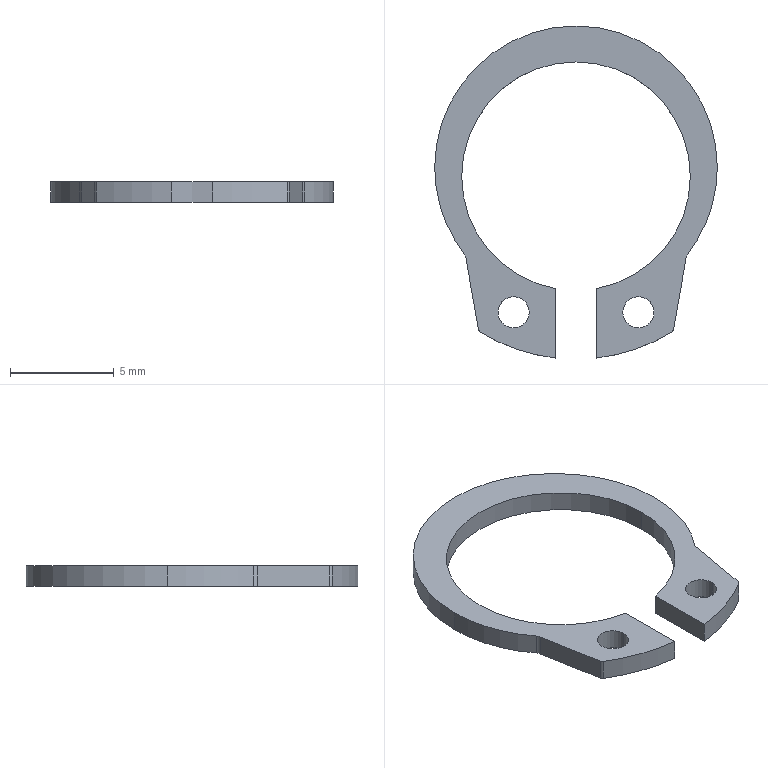Component | SolidWorks | circlips for shaft--type a large gb-1 | 1 solid | 22 faces | box 13.6 x 15.97 x 1 mm | volume 66 mm3 | cylinder 16 | plane 6 | commonest cylinder face diameters 1.5 x4 13.6 x3 11 x3 17.6 x2 0.4 x2 1 x2
build123d program:
from build123d import *

# Parameters (mm, degrees)
SKETCH1_R  = 0.75
BODY_DEPTH = 1
FILLET1_R  = 0.2
FILLET2_R  = 0.5


with BuildPart() as part:
    # Sketch1 → Body (new body)
    with BuildSketch(Plane.XY):
        with BuildLine():
            Line((-1, -5.838), (-1, -9.173))
            ThreePointArc((-1, -9.173), (-2.911, -8.734), (-4.678, -7.884))
            Line((-4.678, -7.884), (-5.322, -4.233))
            ThreePointArc((-5.322, -4.233), (0, 6.8), (5.322, -4.233))
            Line((5.322, -4.233), (4.678, -7.884))
            ThreePointArc((4.678, -7.884), (2.911, -8.734), (1, -9.173))
            Line((1, -9.173), (1, -5.838))
            ThreePointArc((1, -5.838), (0, 5.07), (-1, -5.838))
        make_face()
        with Locations(Location((3, -6.975, 0), (0, 0, 180))):
            Circle(SKETCH1_R, mode=Mode.SUBTRACT)
        with Locations((-3, -6.975)):
            Circle(SKETCH1_R, mode=Mode.SUBTRACT)
    extrude(amount=-BODY_DEPTH)

    # Fillet1
    fillet1_edges = [part.edges().sort_by_distance(p)[0] for p in [
        (-4.678, -7.884, -0.5),
        (4.678, -7.884, -0.5),
    ]]
    fillet(fillet1_edges, radius=FILLET1_R)

    # Fillet2
    fillet2_edges = [part.edges().sort_by_distance(p)[0] for p in [
        (-5.322, -4.233, -0.5),
        (5.322, -4.233, -0.5),
    ]]
    fillet(fillet2_edges, radius=FILLET2_R)


solid = part.part

# Placed as in the assembly
solid = solid.moved(Location((29.5, 189.93, 162), (0, 0, 0)))
STEP:
#1=COLOUR_RGB('',0.7922,0.8196,0.9333);
#2=FILL_AREA_STYLE_COLOUR('',#1);
#3=FILL_AREA_STYLE('',(#2));
#4=SURFACE_STYLE_FILL_AREA(#3);
#5=SURFACE_SIDE_STYLE('',(#4));
#6=SURFACE_STYLE_USAGE(.BOTH.,#5);
#7=PRESENTATION_STYLE_ASSIGNMENT((#6));
#8=CARTESIAN_POINT('',(1.25,7.203,6.339));
#9=VERTEX_POINT('',#8);
#10=CARTESIAN_POINT('',(1.309,7.203,6.339));
#11=VERTEX_POINT('',#10);
#12=CARTESIAN_POINT('',(1.28,7.203,6.339));
#13=DIRECTION('',(0.,0.,1.));
#14=DIRECTION('',(-1.,0.,0.));
#15=AXIS2_PLACEMENT_3D('',#12,#13,#14);
#16=CIRCLE('',#15,0.02953);
#17=EDGE_CURVE('',#9,#11,#16,.T.);
#18=ORIENTED_EDGE('',*,*,#17,.F.);
#19=CARTESIAN_POINT('',(1.25,7.203,6.378));
#20=VERTEX_POINT('',#19);
#21=CARTESIAN_POINT('',(1.25,7.203,6.339));
#22=DIRECTION('',(0.,0.,1.));
#23=VECTOR('',#22,39.37);
#24=LINE('',#21,#23);
#25=EDGE_CURVE('',#9,#20,#24,.T.);
#26=ORIENTED_EDGE('',*,*,#25,.T.);
#27=CARTESIAN_POINT('',(1.309,7.203,6.378));
#28=VERTEX_POINT('',#27);
#29=CARTESIAN_POINT('',(1.28,7.203,6.378));
#30=DIRECTION('',(0.,0.,1.));
#31=DIRECTION('',(-1.,0.,0.));
#32=AXIS2_PLACEMENT_3D('',#29,#30,#31);
#33=CIRCLE('',#32,0.02953);
#34=EDGE_CURVE('',#20,#28,#33,.T.);
#35=ORIENTED_EDGE('',*,*,#34,.T.);
#36=CARTESIAN_POINT('',(1.309,7.203,6.339));
#37=DIRECTION('',(0.,0.,1.));
#38=VECTOR('',#37,39.37);
#39=LINE('',#36,#38);
#40=EDGE_CURVE('',#11,#28,#39,.T.);
#41=ORIENTED_EDGE('',*,*,#40,.F.);
#42=EDGE_LOOP('',(#18,#26,#35,#41));
#43=FACE_OUTER_BOUND('',#42,.T.);
#44=CARTESIAN_POINT('',(1.28,7.203,6.339));
#45=DIRECTION('',(0.,0.,1.));
#46=DIRECTION('',(1.,0.,0.));
#47=AXIS2_PLACEMENT_3D('',#44,#45,#46);
#48=CYLINDRICAL_SURFACE('',#47,0.02953);
#49=ADVANCED_FACE('',(#43),#48,.F.);
#50=CARTESIAN_POINT('',(1.014,7.203,6.339));
#51=VERTEX_POINT('',#50);
#52=CARTESIAN_POINT('',(1.073,7.203,6.339));
#53=VERTEX_POINT('',#52);
#54=CARTESIAN_POINT('',(1.043,7.203,6.339));
#55=DIRECTION('',(0.,0.,1.));
#56=DIRECTION('',(1.,0.,0.));
#57=AXIS2_PLACEMENT_3D('',#54,#55,#56);
#58=CIRCLE('',#57,0.02953);
#59=EDGE_CURVE('',#51,#53,#58,.T.);
#60=ORIENTED_EDGE('',*,*,#59,.F.);
#61=CARTESIAN_POINT('',(1.014,7.203,6.378));
#62=VERTEX_POINT('',#61);
#63=CARTESIAN_POINT('',(1.014,7.203,6.339));
#64=DIRECTION('',(0.,0.,1.));
#65=VECTOR('',#64,39.37);
#66=LINE('',#63,#65);
#67=EDGE_CURVE('',#51,#62,#66,.T.);
#68=ORIENTED_EDGE('',*,*,#67,.T.);
#69=CARTESIAN_POINT('',(1.073,7.203,6.378));
#70=VERTEX_POINT('',#69);
#71=CARTESIAN_POINT('',(1.043,7.203,6.378));
#72=DIRECTION('',(0.,0.,1.));
#73=DIRECTION('',(1.,0.,0.));
#74=AXIS2_PLACEMENT_3D('',#71,#72,#73);
#75=CIRCLE('',#74,0.02953);
#76=EDGE_CURVE('',#62,#70,#75,.T.);
#77=ORIENTED_EDGE('',*,*,#76,.T.);
#78=CARTESIAN_POINT('',(1.073,7.203,6.339));
#79=DIRECTION('',(0.,0.,1.));
#80=VECTOR('',#79,39.37);
#81=LINE('',#78,#80);
#82=EDGE_CURVE('',#53,#70,#81,.T.);
#83=ORIENTED_EDGE('',*,*,#82,.F.);
#84=EDGE_LOOP('',(#60,#68,#77,#83));
#85=FACE_OUTER_BOUND('',#84,.T.);
#86=CARTESIAN_POINT('',(1.043,7.203,6.339));
#87=DIRECTION('',(0.,0.,1.));
#88=DIRECTION('',(1.,0.,0.));
#89=AXIS2_PLACEMENT_3D('',#86,#87,#88);
#90=CYLINDRICAL_SURFACE('',#89,0.02953);
#91=ADVANCED_FACE('',(#85),#90,.F.);
#92=CARTESIAN_POINT('',(1.429,7.478,6.339));
#93=VERTEX_POINT('',#92);
#94=CARTESIAN_POINT('',(0.8937,7.478,6.339));
#95=VERTEX_POINT('',#94);
#96=CARTESIAN_POINT('',(1.161,7.478,6.339));
#97=DIRECTION('',(0.,0.,1.));
#98=DIRECTION('',(1.,0.,0.));
#99=AXIS2_PLACEMENT_3D('',#96,#97,#98);
#100=CIRCLE('',#99,0.2677);
#101=EDGE_CURVE('',#93,#95,#100,.T.);
#102=ORIENTED_EDGE('',*,*,#101,.T.);
#103=CARTESIAN_POINT('',(0.8937,7.478,6.378));
#104=VERTEX_POINT('',#103);
#105=CARTESIAN_POINT('',(0.8937,7.478,6.339));
#106=DIRECTION('',(0.,0.,1.));
#107=VECTOR('',#106,39.37);
#108=LINE('',#105,#107);
#109=EDGE_CURVE('',#95,#104,#108,.T.);
#110=ORIENTED_EDGE('',*,*,#109,.T.);
#111=CARTESIAN_POINT('',(1.429,7.478,6.378));
#112=VERTEX_POINT('',#111);
#113=CARTESIAN_POINT('',(1.161,7.478,6.378));
#114=DIRECTION('',(0.,0.,1.));
#115=DIRECTION('',(1.,0.,0.));
#116=AXIS2_PLACEMENT_3D('',#113,#114,#115);
#117=CIRCLE('',#116,0.2677);
#118=EDGE_CURVE('',#112,#104,#117,.T.);
#119=ORIENTED_EDGE('',*,*,#118,.F.);
#120=CARTESIAN_POINT('',(1.429,7.478,6.339));
#121=DIRECTION('',(0.,0.,1.));
#122=VECTOR('',#121,39.37);
#123=LINE('',#120,#122);
#124=EDGE_CURVE('',#93,#112,#123,.T.);
#125=ORIENTED_EDGE('',*,*,#124,.F.);
#126=EDGE_LOOP('',(#102,#110,#119,#125));
#127=FACE_OUTER_BOUND('',#126,.T.);
#128=CARTESIAN_POINT('',(1.161,7.478,6.339));
#129=DIRECTION('',(0.,0.,1.));
#130=DIRECTION('',(1.,0.,0.));
#131=AXIS2_PLACEMENT_3D('',#128,#129,#130);
#132=CYLINDRICAL_SURFACE('',#131,0.2677);
#133=ADVANCED_FACE('',(#127),#132,.T.);
#134=CARTESIAN_POINT('',(1.374,7.315,6.339));
#135=VERTEX_POINT('',#134);
#136=CARTESIAN_POINT('',(1.161,7.478,6.339));
#137=DIRECTION('',(0.,0.,1.));
#138=DIRECTION('',(1.,0.,0.));
#139=AXIS2_PLACEMENT_3D('',#136,#137,#138);
#140=CIRCLE('',#139,0.2677);
#141=EDGE_CURVE('',#135,#93,#140,.T.);
#142=ORIENTED_EDGE('',*,*,#141,.T.);
#143=ORIENTED_EDGE('',*,*,#124,.T.);
#144=CARTESIAN_POINT('',(1.374,7.315,6.378));
#145=VERTEX_POINT('',#144);
#146=CARTESIAN_POINT('',(1.161,7.478,6.378));
#147=DIRECTION('',(0.,0.,1.));
#148=DIRECTION('',(1.,0.,0.));
#149=AXIS2_PLACEMENT_3D('',#146,#147,#148);
#150=CIRCLE('',#149,0.2677);
#151=EDGE_CURVE('',#145,#112,#150,.T.);
#152=ORIENTED_EDGE('',*,*,#151,.F.);
#153=CARTESIAN_POINT('',(1.374,7.315,6.339));
#154=DIRECTION('',(0.,0.,-1.));
#155=VECTOR('',#154,39.37);
#156=LINE('',#153,#155);
#157=EDGE_CURVE('',#145,#135,#156,.T.);
#158=ORIENTED_EDGE('',*,*,#157,.T.);
#159=EDGE_LOOP('',(#142,#143,#152,#158));
#160=FACE_OUTER_BOUND('',#159,.T.);
#161=CARTESIAN_POINT('',(1.161,7.478,6.339));
#162=DIRECTION('',(0.,0.,1.));
#163=DIRECTION('',(1.,0.,0.));
#164=AXIS2_PLACEMENT_3D('',#161,#162,#163);
#165=CYLINDRICAL_SURFACE('',#164,0.2677);
#166=ADVANCED_FACE('',(#160),#165,.T.);
#167=CARTESIAN_POINT('',(1.122,7.248,6.339));
#168=VERTEX_POINT('',#167);
#169=CARTESIAN_POINT('',(0.9449,7.461,6.339));
#170=VERTEX_POINT('',#169);
#171=CARTESIAN_POINT('',(1.161,7.461,6.339));
#172=DIRECTION('',(0.,0.,-1.));
#173=DIRECTION('',(1.,0.,0.));
#174=AXIS2_PLACEMENT_3D('',#171,#172,#173);
#175=CIRCLE('',#174,0.2165);
#176=EDGE_CURVE('',#168,#170,#175,.T.);
#177=ORIENTED_EDGE('',*,*,#176,.T.);
#178=CARTESIAN_POINT('',(0.9449,7.461,6.378));
#179=VERTEX_POINT('',#178);
#180=CARTESIAN_POINT('',(0.9449,7.461,6.339));
#181=DIRECTION('',(0.,0.,1.));
#182=VECTOR('',#181,39.37);
#183=LINE('',#180,#182);
#184=EDGE_CURVE('',#170,#179,#183,.T.);
#185=ORIENTED_EDGE('',*,*,#184,.T.);
#186=CARTESIAN_POINT('',(1.122,7.248,6.378));
#187=VERTEX_POINT('',#186);
#188=CARTESIAN_POINT('',(1.161,7.461,6.378));
#189=DIRECTION('',(0.,0.,-1.));
#190=DIRECTION('',(1.,0.,0.));
#191=AXIS2_PLACEMENT_3D('',#188,#189,#190);
#192=CIRCLE('',#191,0.2165);
#193=EDGE_CURVE('',#187,#179,#192,.T.);
#194=ORIENTED_EDGE('',*,*,#193,.F.);
#195=CARTESIAN_POINT('',(1.122,7.248,6.339));
#196=DIRECTION('',(0.,0.,1.));
#197=VECTOR('',#196,39.37);
#198=LINE('',#195,#197);
#199=EDGE_CURVE('',#168,#187,#198,.T.);
#200=ORIENTED_EDGE('',*,*,#199,.F.);
#201=EDGE_LOOP('',(#177,#185,#194,#200));
#202=FACE_OUTER_BOUND('',#201,.T.);
#203=CARTESIAN_POINT('',(1.161,7.461,6.339));
#204=DIRECTION('',(0.,0.,1.));
#205=DIRECTION('',(1.,0.,0.));
#206=AXIS2_PLACEMENT_3D('',#203,#204,#205);
#207=CYLINDRICAL_SURFACE('',#206,0.2165);
#208=ADVANCED_FACE('',(#202),#207,.F.);
#209=ORIENTED_EDGE('',*,*,#184,.F.);
#210=CARTESIAN_POINT('',(1.378,7.461,6.339));
#211=VERTEX_POINT('',#210);
#212=CARTESIAN_POINT('',(1.161,7.461,6.339));
#213=DIRECTION('',(0.,0.,-1.));
#214=DIRECTION('',(1.,0.,0.));
#215=AXIS2_PLACEMENT_3D('',#212,#213,#214);
#216=CIRCLE('',#215,0.2165);
#217=EDGE_CURVE('',#170,#211,#216,.T.);
#218=ORIENTED_EDGE('',*,*,#217,.T.);
#219=CARTESIAN_POINT('',(1.378,7.461,6.378));
#220=VERTEX_POINT('',#219);
#221=CARTESIAN_POINT('',(1.378,7.461,6.339));
#222=DIRECTION('',(0.,0.,1.));
#223=VECTOR('',#222,39.37);
#224=LINE('',#221,#223);
#225=EDGE_CURVE('',#211,#220,#224,.T.);
#226=ORIENTED_EDGE('',*,*,#225,.T.);
#227=CARTESIAN_POINT('',(1.161,7.461,6.378));
#228=DIRECTION('',(0.,0.,-1.));
#229=DIRECTION('',(1.,0.,0.));
#230=AXIS2_PLACEMENT_3D('',#227,#228,#229);
#231=CIRCLE('',#230,0.2165);
#232=EDGE_CURVE('',#179,#220,#231,.T.);
#233=ORIENTED_EDGE('',*,*,#232,.F.);
#234=EDGE_LOOP('',(#209,#218,#226,#233));
#235=FACE_OUTER_BOUND('',#234,.T.);
#236=CARTESIAN_POINT('',(1.161,7.461,6.339));
#237=DIRECTION('',(0.,0.,1.));
#238=DIRECTION('',(1.,0.,0.));
#239=AXIS2_PLACEMENT_3D('',#236,#237,#238);
#240=CYLINDRICAL_SURFACE('',#239,0.2165);
#241=ADVANCED_FACE('',(#235),#240,.F.);
#242=CARTESIAN_POINT('',(1.201,7.116,6.339));
#243=VERTEX_POINT('',#242);
#244=CARTESIAN_POINT('',(1.343,7.165,6.339));
#245=VERTEX_POINT('',#244);
#246=CARTESIAN_POINT('',(1.161,7.461,6.339));
#247=DIRECTION('',(0.,0.,1.));
#248=DIRECTION('',(-1.,0.,0.));
#249=AXIS2_PLACEMENT_3D('',#246,#247,#248);
#250=CIRCLE('',#249,0.3465);
#251=EDGE_CURVE('',#243,#245,#250,.T.);
#252=ORIENTED_EDGE('',*,*,#251,.T.);
#253=CARTESIAN_POINT('',(1.343,7.165,6.378));
#254=VERTEX_POINT('',#253);
#255=CARTESIAN_POINT('',(1.343,7.165,6.339));
#256=DIRECTION('',(0.,0.,1.));
#257=VECTOR('',#256,39.37);
#258=LINE('',#255,#257);
#259=EDGE_CURVE('',#245,#254,#258,.T.);
#260=ORIENTED_EDGE('',*,*,#259,.T.);
#261=CARTESIAN_POINT('',(1.201,7.116,6.378));
#262=VERTEX_POINT('',#261);
#263=CARTESIAN_POINT('',(1.161,7.461,6.378));
#264=DIRECTION('',(0.,0.,1.));
#265=DIRECTION('',(-1.,0.,0.));
#266=AXIS2_PLACEMENT_3D('',#263,#264,#265);
#267=CIRCLE('',#266,0.3465);
#268=EDGE_CURVE('',#262,#254,#267,.T.);
#269=ORIENTED_EDGE('',*,*,#268,.F.);
#270=CARTESIAN_POINT('',(1.201,7.116,6.339));
#271=DIRECTION('',(0.,0.,1.));
#272=VECTOR('',#271,39.37);
#273=LINE('',#270,#272);
#274=EDGE_CURVE('',#243,#262,#273,.T.);
#275=ORIENTED_EDGE('',*,*,#274,.F.);
#276=EDGE_LOOP('',(#252,#260,#269,#275));
#277=FACE_OUTER_BOUND('',#276,.T.);
#278=CARTESIAN_POINT('',(1.161,7.461,6.339));
#279=DIRECTION('',(0.,0.,1.));
#280=DIRECTION('',(1.,0.,0.));
#281=AXIS2_PLACEMENT_3D('',#278,#279,#280);
#282=CYLINDRICAL_SURFACE('',#281,0.3465);
#283=ADVANCED_FACE('',(#277),#282,.T.);
#284=CARTESIAN_POINT('',(1.201,7.248,6.378));
#285=VERTEX_POINT('',#284);
#286=CARTESIAN_POINT('',(1.201,7.248,6.378));
#287=DIRECTION('',(0.,-1.,0.));
#288=VECTOR('',#287,39.37);
#289=LINE('',#286,#288);
#290=EDGE_CURVE('',#285,#262,#289,.T.);
#291=ORIENTED_EDGE('',*,*,#290,.F.);
#292=CARTESIAN_POINT('',(1.201,7.248,6.339));
#293=VERTEX_POINT('',#292);
#294=CARTESIAN_POINT('',(1.201,7.248,6.339));
#295=DIRECTION('',(0.,0.,1.));
#296=VECTOR('',#295,39.37);
#297=LINE('',#294,#296);
#298=EDGE_CURVE('',#293,#285,#297,.T.);
#299=ORIENTED_EDGE('',*,*,#298,.F.);
#300=CARTESIAN_POINT('',(1.201,7.248,6.339));
#301=DIRECTION('',(0.,-1.,0.));
#302=VECTOR('',#301,39.37);
#303=LINE('',#300,#302);
#304=EDGE_CURVE('',#293,#243,#303,.T.);
#305=ORIENTED_EDGE('',*,*,#304,.T.);
#306=ORIENTED_EDGE('',*,*,#274,.T.);
#307=EDGE_LOOP('',(#291,#299,#305,#306));
#308=FACE_OUTER_BOUND('',#307,.T.);
#309=CARTESIAN_POINT('',(1.201,7.248,6.339));
#310=DIRECTION('',(-1.,-0.,0.));
#311=DIRECTION('',(0.,-1.,0.));
#312=AXIS2_PLACEMENT_3D('',#309,#310,#311);
#313=PLANE('',#312);
#314=ADVANCED_FACE('',(#308),#313,.T.);
#315=ORIENTED_EDGE('',*,*,#225,.F.);
#316=CARTESIAN_POINT('',(1.161,7.461,6.339));
#317=DIRECTION('',(0.,0.,-1.));
#318=DIRECTION('',(1.,0.,0.));
#319=AXIS2_PLACEMENT_3D('',#316,#317,#318);
#320=CIRCLE('',#319,0.2165);
#321=EDGE_CURVE('',#211,#293,#320,.T.);
#322=ORIENTED_EDGE('',*,*,#321,.T.);
#323=ORIENTED_EDGE('',*,*,#298,.T.);
#324=CARTESIAN_POINT('',(1.161,7.461,6.378));
#325=DIRECTION('',(0.,0.,-1.));
#326=DIRECTION('',(1.,0.,0.));
#327=AXIS2_PLACEMENT_3D('',#324,#325,#326);
#328=CIRCLE('',#327,0.2165);
#329=EDGE_CURVE('',#220,#285,#328,.T.);
#330=ORIENTED_EDGE('',*,*,#329,.F.);
#331=EDGE_LOOP('',(#315,#322,#323,#330));
#332=FACE_OUTER_BOUND('',#331,.T.);
#333=CARTESIAN_POINT('',(1.161,7.461,6.339));
#334=DIRECTION('',(0.,0.,1.));
#335=DIRECTION('',(1.,0.,0.));
#336=AXIS2_PLACEMENT_3D('',#333,#334,#335);
#337=CYLINDRICAL_SURFACE('',#336,0.2165);
#338=ADVANCED_FACE('',(#332),#337,.F.);
#339=CARTESIAN_POINT('',(1.122,7.116,6.378));
#340=VERTEX_POINT('',#339);
#341=CARTESIAN_POINT('',(1.122,7.248,6.378));
#342=DIRECTION('',(0.,1.,0.));
#343=VECTOR('',#342,39.37);
#344=LINE('',#341,#343);
#345=EDGE_CURVE('',#340,#187,#344,.T.);
#346=ORIENTED_EDGE('',*,*,#345,.F.);
#347=CARTESIAN_POINT('',(1.122,7.116,6.339));
#348=VERTEX_POINT('',#347);
#349=CARTESIAN_POINT('',(1.122,7.116,6.339));
#350=DIRECTION('',(0.,0.,1.));
#351=VECTOR('',#350,39.37);
#352=LINE('',#349,#351);
#353=EDGE_CURVE('',#348,#340,#352,.T.);
#354=ORIENTED_EDGE('',*,*,#353,.F.);
#355=CARTESIAN_POINT('',(1.122,7.248,6.339));
#356=DIRECTION('',(0.,1.,0.));
#357=VECTOR('',#356,39.37);
#358=LINE('',#355,#357);
#359=EDGE_CURVE('',#348,#168,#358,.T.);
#360=ORIENTED_EDGE('',*,*,#359,.T.);
#361=ORIENTED_EDGE('',*,*,#199,.T.);
#362=EDGE_LOOP('',(#346,#354,#360,#361));
#363=FACE_OUTER_BOUND('',#362,.T.);
#364=CARTESIAN_POINT('',(1.122,7.248,6.339));
#365=DIRECTION('',(1.,-0.,0.));
#366=DIRECTION('',(0.,1.,0.));
#367=AXIS2_PLACEMENT_3D('',#364,#365,#366);
#368=PLANE('',#367);
#369=ADVANCED_FACE('',(#363),#368,.T.);
#370=CARTESIAN_POINT('',(0.9803,7.165,6.378));
#371=VERTEX_POINT('',#370);
#372=CARTESIAN_POINT('',(1.161,7.461,6.378));
#373=DIRECTION('',(0.,0.,1.));
#374=DIRECTION('',(1.,0.,0.));
#375=AXIS2_PLACEMENT_3D('',#372,#373,#374);
#376=CIRCLE('',#375,0.3465);
#377=EDGE_CURVE('',#371,#340,#376,.T.);
#378=ORIENTED_EDGE('',*,*,#377,.F.);
#379=CARTESIAN_POINT('',(0.9803,7.165,6.339));
#380=VERTEX_POINT('',#379);
#381=CARTESIAN_POINT('',(0.9803,7.165,6.339));
#382=DIRECTION('',(0.,0.,-1.));
#383=VECTOR('',#382,39.37);
#384=LINE('',#381,#383);
#385=EDGE_CURVE('',#371,#380,#384,.T.);
#386=ORIENTED_EDGE('',*,*,#385,.T.);
#387=CARTESIAN_POINT('',(1.161,7.461,6.339));
#388=DIRECTION('',(0.,0.,1.));
#389=DIRECTION('',(1.,0.,0.));
#390=AXIS2_PLACEMENT_3D('',#387,#388,#389);
#391=CIRCLE('',#390,0.3465);
#392=EDGE_CURVE('',#380,#348,#391,.T.);
#393=ORIENTED_EDGE('',*,*,#392,.T.);
#394=ORIENTED_EDGE('',*,*,#353,.T.);
#395=EDGE_LOOP('',(#378,#386,#393,#394));
#396=FACE_OUTER_BOUND('',#395,.T.);
#397=CARTESIAN_POINT('',(1.161,7.461,6.339));
#398=DIRECTION('',(0.,0.,1.));
#399=DIRECTION('',(1.,0.,0.));
#400=AXIS2_PLACEMENT_3D('',#397,#398,#399);
#401=CYLINDRICAL_SURFACE('',#400,0.3465);
#402=ADVANCED_FACE('',(#396),#401,.T.);
#403=CARTESIAN_POINT('',(0.9527,7.306,6.378));
#404=VERTEX_POINT('',#403);
#405=CARTESIAN_POINT('',(0.9766,7.171,6.378));
#406=VERTEX_POINT('',#405);
#407=CARTESIAN_POINT('',(0.9519,7.311,6.378));
#408=DIRECTION('',(0.1736,-0.9848,0.));
#409=VECTOR('',#408,39.37);
#410=LINE('',#407,#409);
#411=EDGE_CURVE('',#404,#406,#410,.T.);
#412=ORIENTED_EDGE('',*,*,#411,.F.);
#413=CARTESIAN_POINT('',(0.9527,7.306,6.339));
#414=VERTEX_POINT('',#413);
#415=CARTESIAN_POINT('',(0.9527,7.306,6.339));
#416=DIRECTION('',(0.,0.,-1.));
#417=VECTOR('',#416,39.37);
#418=LINE('',#415,#417);
#419=EDGE_CURVE('',#404,#414,#418,.T.);
#420=ORIENTED_EDGE('',*,*,#419,.T.);
#421=CARTESIAN_POINT('',(0.9766,7.171,6.339));
#422=VERTEX_POINT('',#421);
#423=CARTESIAN_POINT('',(0.9519,7.311,6.339));
#424=DIRECTION('',(0.1736,-0.9848,0.));
#425=VECTOR('',#424,39.37);
#426=LINE('',#423,#425);
#427=EDGE_CURVE('',#414,#422,#426,.T.);
#428=ORIENTED_EDGE('',*,*,#427,.T.);
#429=CARTESIAN_POINT('',(0.9766,7.171,6.339));
#430=DIRECTION('',(0.,0.,1.));
#431=VECTOR('',#430,39.37);
#432=LINE('',#429,#431);
#433=EDGE_CURVE('',#422,#406,#432,.T.);
#434=ORIENTED_EDGE('',*,*,#433,.T.);
#435=EDGE_LOOP('',(#412,#420,#428,#434));
#436=FACE_OUTER_BOUND('',#435,.T.);
#437=CARTESIAN_POINT('',(0.9519,7.311,6.339));
#438=DIRECTION('',(-0.9848,-0.1736,0.));
#439=DIRECTION('',(0.1736,-0.9848,0.));
#440=AXIS2_PLACEMENT_3D('',#437,#438,#439);
#441=PLANE('',#440);
#442=ADVANCED_FACE('',(#436),#441,.T.);
#443=ORIENTED_EDGE('',*,*,#109,.F.);
#444=CARTESIAN_POINT('',(0.949,7.315,6.339));
#445=VERTEX_POINT('',#444);
#446=CARTESIAN_POINT('',(1.161,7.478,6.339));
#447=DIRECTION('',(0.,0.,1.));
#448=DIRECTION('',(1.,0.,0.));
#449=AXIS2_PLACEMENT_3D('',#446,#447,#448);
#450=CIRCLE('',#449,0.2677);
#451=EDGE_CURVE('',#95,#445,#450,.T.);
#452=ORIENTED_EDGE('',*,*,#451,.T.);
#453=CARTESIAN_POINT('',(0.949,7.315,6.378));
#454=VERTEX_POINT('',#453);
#455=CARTESIAN_POINT('',(0.949,7.315,6.339));
#456=DIRECTION('',(0.,0.,1.));
#457=VECTOR('',#456,39.37);
#458=LINE('',#455,#457);
#459=EDGE_CURVE('',#445,#454,#458,.T.);
#460=ORIENTED_EDGE('',*,*,#459,.T.);
#461=CARTESIAN_POINT('',(1.161,7.478,6.378));
#462=DIRECTION('',(0.,0.,1.));
#463=DIRECTION('',(1.,0.,0.));
#464=AXIS2_PLACEMENT_3D('',#461,#462,#463);
#465=CIRCLE('',#464,0.2677);
#466=EDGE_CURVE('',#104,#454,#465,.T.);
#467=ORIENTED_EDGE('',*,*,#466,.F.);
#468=EDGE_LOOP('',(#443,#452,#460,#467));
#469=FACE_OUTER_BOUND('',#468,.T.);
#470=CARTESIAN_POINT('',(1.161,7.478,6.339));
#471=DIRECTION('',(0.,0.,1.));
#472=DIRECTION('',(1.,0.,0.));
#473=AXIS2_PLACEMENT_3D('',#470,#471,#472);
#474=CYLINDRICAL_SURFACE('',#473,0.2677);
#475=ADVANCED_FACE('',(#469),#474,.T.);
#476=CARTESIAN_POINT('',(1.346,7.171,6.339));
#477=VERTEX_POINT('',#476);
#478=CARTESIAN_POINT('',(1.37,7.306,6.339));
#479=VERTEX_POINT('',#478);
#480=CARTESIAN_POINT('',(1.371,7.311,6.339));
#481=DIRECTION('',(0.1736,0.9848,0.));
#482=VECTOR('',#481,39.37);
#483=LINE('',#480,#482);
#484=EDGE_CURVE('',#477,#479,#483,.T.);
#485=ORIENTED_EDGE('',*,*,#484,.T.);
#486=CARTESIAN_POINT('',(1.37,7.306,6.378));
#487=VERTEX_POINT('',#486);
#488=CARTESIAN_POINT('',(1.37,7.306,6.378));
#489=DIRECTION('',(0.,0.,1.));
#490=VECTOR('',#489,39.37);
#491=LINE('',#488,#490);
#492=EDGE_CURVE('',#479,#487,#491,.T.);
#493=ORIENTED_EDGE('',*,*,#492,.T.);
#494=CARTESIAN_POINT('',(1.346,7.171,6.378));
#495=VERTEX_POINT('',#494);
#496=CARTESIAN_POINT('',(1.371,7.311,6.378));
#497=DIRECTION('',(0.1736,0.9848,0.));
#498=VECTOR('',#497,39.37);
#499=LINE('',#496,#498);
#500=EDGE_CURVE('',#495,#487,#499,.T.);
#501=ORIENTED_EDGE('',*,*,#500,.F.);
#502=CARTESIAN_POINT('',(1.346,7.171,6.339));
#503=DIRECTION('',(0.,0.,-1.));
#504=VECTOR('',#503,39.37);
#505=LINE('',#502,#504);
#506=EDGE_CURVE('',#495,#477,#505,.T.);
#507=ORIENTED_EDGE('',*,*,#506,.T.);
#508=EDGE_LOOP('',(#485,#493,#501,#507));
#509=FACE_OUTER_BOUND('',#508,.T.);
#510=CARTESIAN_POINT('',(1.371,7.311,6.339));
#511=DIRECTION('',(0.9848,-0.1736,0.));
#512=DIRECTION('',(0.1736,0.9848,0.));
#513=AXIS2_PLACEMENT_3D('',#510,#511,#512);
#514=PLANE('',#513);
#515=ADVANCED_FACE('',(#509),#514,.T.);
#516=CARTESIAN_POINT('',(1.28,7.203,6.339));
#517=DIRECTION('',(0.,0.,1.));
#518=DIRECTION('',(-1.,0.,0.));
#519=AXIS2_PLACEMENT_3D('',#516,#517,#518);
#520=CIRCLE('',#519,0.02953);
#521=EDGE_CURVE('',#11,#9,#520,.T.);
#522=ORIENTED_EDGE('',*,*,#521,.T.);
#523=ORIENTED_EDGE('',*,*,#17,.T.);
#524=EDGE_LOOP('',(#522,#523));
#525=FACE_BOUND('',#524,.T.);
#526=CARTESIAN_POINT('',(1.043,7.203,6.339));
#527=DIRECTION('',(0.,0.,1.));
#528=DIRECTION('',(1.,0.,0.));
#529=AXIS2_PLACEMENT_3D('',#526,#527,#528);
#530=CIRCLE('',#529,0.02953);
#531=EDGE_CURVE('',#53,#51,#530,.T.);
#532=ORIENTED_EDGE('',*,*,#531,.T.);
#533=ORIENTED_EDGE('',*,*,#59,.T.);
#534=EDGE_LOOP('',(#532,#533));
#535=FACE_BOUND('',#534,.T.);
#536=ORIENTED_EDGE('',*,*,#392,.F.);
#537=CARTESIAN_POINT('',(0.9844,7.172,6.339));
#538=DIRECTION('',(0.,0.,-1.));
#539=DIRECTION('',(-1.,0.,0.));
#540=AXIS2_PLACEMENT_3D('',#537,#538,#539);
#541=CIRCLE('',#540,0.007874);
#542=EDGE_CURVE('',#380,#422,#541,.T.);
#543=ORIENTED_EDGE('',*,*,#542,.T.);
#544=ORIENTED_EDGE('',*,*,#427,.F.);
#545=CARTESIAN_POINT('',(0.9334,7.303,6.339));
#546=DIRECTION('',(0.,0.,1.));
#547=DIRECTION('',(-1.,-0.,0.));
#548=AXIS2_PLACEMENT_3D('',#545,#546,#547);
#549=CIRCLE('',#548,0.01969);
#550=EDGE_CURVE('',#414,#445,#549,.T.);
#551=ORIENTED_EDGE('',*,*,#550,.T.);
#552=ORIENTED_EDGE('',*,*,#451,.F.);
#553=ORIENTED_EDGE('',*,*,#101,.F.);
#554=ORIENTED_EDGE('',*,*,#141,.F.);
#555=CARTESIAN_POINT('',(1.389,7.303,6.339));
#556=DIRECTION('',(0.,0.,1.));
#557=DIRECTION('',(-1.,-0.,0.));
#558=AXIS2_PLACEMENT_3D('',#555,#556,#557);
#559=CIRCLE('',#558,0.01969);
#560=EDGE_CURVE('',#135,#479,#559,.T.);
#561=ORIENTED_EDGE('',*,*,#560,.T.);
#562=ORIENTED_EDGE('',*,*,#484,.F.);
#563=CARTESIAN_POINT('',(1.338,7.172,6.339));
#564=DIRECTION('',(0.,0.,-1.));
#565=DIRECTION('',(-1.,0.,0.));
#566=AXIS2_PLACEMENT_3D('',#563,#564,#565);
#567=CIRCLE('',#566,0.007874);
#568=EDGE_CURVE('',#477,#245,#567,.T.);
#569=ORIENTED_EDGE('',*,*,#568,.T.);
#570=ORIENTED_EDGE('',*,*,#251,.F.);
#571=ORIENTED_EDGE('',*,*,#304,.F.);
#572=ORIENTED_EDGE('',*,*,#321,.F.);
#573=ORIENTED_EDGE('',*,*,#217,.F.);
#574=ORIENTED_EDGE('',*,*,#176,.F.);
#575=ORIENTED_EDGE('',*,*,#359,.F.);
#576=EDGE_LOOP('',(#536,#543,#544,#551,#552,#553,#554,#561,#562,#569,#570,#571,#572,#573,#574,#575));
#577=FACE_OUTER_BOUND('',#576,.T.);
#578=CARTESIAN_POINT('',(1.161,7.461,6.339));
#579=DIRECTION('',(0.,0.,-1.));
#580=DIRECTION('',(-1.,0.,0.));
#581=AXIS2_PLACEMENT_3D('',#578,#579,#580);
#582=PLANE('',#581);
#583=ADVANCED_FACE('',(#525,#535,#577),#582,.T.);
#584=CARTESIAN_POINT('',(1.28,7.203,6.378));
#585=DIRECTION('',(0.,0.,1.));
#586=DIRECTION('',(-1.,0.,0.));
#587=AXIS2_PLACEMENT_3D('',#584,#585,#586);
#588=CIRCLE('',#587,0.02953);
#589=EDGE_CURVE('',#28,#20,#588,.T.);
#590=ORIENTED_EDGE('',*,*,#589,.F.);
#591=ORIENTED_EDGE('',*,*,#34,.F.);
#592=EDGE_LOOP('',(#590,#591));
#593=FACE_BOUND('',#592,.T.);
#594=CARTESIAN_POINT('',(1.043,7.203,6.378));
#595=DIRECTION('',(0.,0.,1.));
#596=DIRECTION('',(1.,0.,0.));
#597=AXIS2_PLACEMENT_3D('',#594,#595,#596);
#598=CIRCLE('',#597,0.02953);
#599=EDGE_CURVE('',#70,#62,#598,.T.);
#600=ORIENTED_EDGE('',*,*,#599,.F.);
#601=ORIENTED_EDGE('',*,*,#76,.F.);
#602=EDGE_LOOP('',(#600,#601));
#603=FACE_BOUND('',#602,.T.);
#604=ORIENTED_EDGE('',*,*,#151,.T.);
#605=ORIENTED_EDGE('',*,*,#118,.T.);
#606=ORIENTED_EDGE('',*,*,#466,.T.);
#607=CARTESIAN_POINT('',(0.9334,7.303,6.378));
#608=DIRECTION('',(0.,0.,-1.));
#609=DIRECTION('',(-1.,0.,0.));
#610=AXIS2_PLACEMENT_3D('',#607,#608,#609);
#611=CIRCLE('',#610,0.01969);
#612=EDGE_CURVE('',#454,#404,#611,.T.);
#613=ORIENTED_EDGE('',*,*,#612,.T.);
#614=ORIENTED_EDGE('',*,*,#411,.T.);
#615=CARTESIAN_POINT('',(0.9844,7.172,6.378));
#616=DIRECTION('',(0.,0.,1.));
#617=DIRECTION('',(-1.,0.,0.));
#618=AXIS2_PLACEMENT_3D('',#615,#616,#617);
#619=CIRCLE('',#618,0.007874);
#620=EDGE_CURVE('',#406,#371,#619,.T.);
#621=ORIENTED_EDGE('',*,*,#620,.T.);
#622=ORIENTED_EDGE('',*,*,#377,.T.);
#623=ORIENTED_EDGE('',*,*,#345,.T.);
#624=ORIENTED_EDGE('',*,*,#193,.T.);
#625=ORIENTED_EDGE('',*,*,#232,.T.);
#626=ORIENTED_EDGE('',*,*,#329,.T.);
#627=ORIENTED_EDGE('',*,*,#290,.T.);
#628=ORIENTED_EDGE('',*,*,#268,.T.);
#629=CARTESIAN_POINT('',(1.338,7.172,6.378));
#630=DIRECTION('',(0.,0.,1.));
#631=DIRECTION('',(-1.,0.,0.));
#632=AXIS2_PLACEMENT_3D('',#629,#630,#631);
#633=CIRCLE('',#632,0.007874);
#634=EDGE_CURVE('',#254,#495,#633,.T.);
#635=ORIENTED_EDGE('',*,*,#634,.T.);
#636=ORIENTED_EDGE('',*,*,#500,.T.);
#637=CARTESIAN_POINT('',(1.389,7.303,6.378));
#638=DIRECTION('',(0.,0.,-1.));
#639=DIRECTION('',(-1.,0.,0.));
#640=AXIS2_PLACEMENT_3D('',#637,#638,#639);
#641=CIRCLE('',#640,0.01969);
#642=EDGE_CURVE('',#487,#145,#641,.T.);
#643=ORIENTED_EDGE('',*,*,#642,.T.);
#644=EDGE_LOOP('',(#604,#605,#606,#613,#614,#621,#622,#623,#624,#625,#626,#627,#628,#635,#636,#643));
#645=FACE_OUTER_BOUND('',#644,.T.);
#646=CARTESIAN_POINT('',(1.161,7.461,6.378));
#647=DIRECTION('',(0.,0.,-1.));
#648=DIRECTION('',(-1.,0.,0.));
#649=AXIS2_PLACEMENT_3D('',#646,#647,#648);
#650=PLANE('',#649);
#651=ADVANCED_FACE('',(#593,#603,#645),#650,.F.);
#652=ORIENTED_EDGE('',*,*,#67,.F.);
#653=ORIENTED_EDGE('',*,*,#531,.F.);
#654=ORIENTED_EDGE('',*,*,#82,.T.);
#655=ORIENTED_EDGE('',*,*,#599,.T.);
#656=EDGE_LOOP('',(#652,#653,#654,#655));
#657=FACE_OUTER_BOUND('',#656,.T.);
#658=CARTESIAN_POINT('',(1.043,7.203,6.339));
#659=DIRECTION('',(0.,0.,1.));
#660=DIRECTION('',(1.,0.,0.));
#661=AXIS2_PLACEMENT_3D('',#658,#659,#660);
#662=CYLINDRICAL_SURFACE('',#661,0.02953);
#663=ADVANCED_FACE('',(#657),#662,.F.);
#664=ORIENTED_EDGE('',*,*,#25,.F.);
#665=ORIENTED_EDGE('',*,*,#521,.F.);
#666=ORIENTED_EDGE('',*,*,#40,.T.);
#667=ORIENTED_EDGE('',*,*,#589,.T.);
#668=EDGE_LOOP('',(#664,#665,#666,#667));
#669=FACE_OUTER_BOUND('',#668,.T.);
#670=CARTESIAN_POINT('',(1.28,7.203,6.339));
#671=DIRECTION('',(0.,0.,1.));
#672=DIRECTION('',(1.,0.,0.));
#673=AXIS2_PLACEMENT_3D('',#670,#671,#672);
#674=CYLINDRICAL_SURFACE('',#673,0.02953);
#675=ADVANCED_FACE('',(#669),#674,.F.);
#676=ORIENTED_EDGE('',*,*,#542,.F.);
#677=ORIENTED_EDGE('',*,*,#385,.F.);
#678=ORIENTED_EDGE('',*,*,#620,.F.);
#679=ORIENTED_EDGE('',*,*,#433,.F.);
#680=EDGE_LOOP('',(#676,#677,#678,#679));
#681=FACE_OUTER_BOUND('',#680,.T.);
#682=CARTESIAN_POINT('',(0.9844,7.172,6.339));
#683=DIRECTION('',(0.,0.,1.));
#684=DIRECTION('',(1.,0.,0.));
#685=AXIS2_PLACEMENT_3D('',#682,#683,#684);
#686=CYLINDRICAL_SURFACE('',#685,0.007874);
#687=ADVANCED_FACE('',(#681),#686,.T.);
#688=ORIENTED_EDGE('',*,*,#568,.F.);
#689=ORIENTED_EDGE('',*,*,#506,.F.);
#690=ORIENTED_EDGE('',*,*,#634,.F.);
#691=ORIENTED_EDGE('',*,*,#259,.F.);
#692=EDGE_LOOP('',(#688,#689,#690,#691));
#693=FACE_OUTER_BOUND('',#692,.T.);
#694=CARTESIAN_POINT('',(1.338,7.172,6.339));
#695=DIRECTION('',(0.,0.,1.));
#696=DIRECTION('',(1.,0.,0.));
#697=AXIS2_PLACEMENT_3D('',#694,#695,#696);
#698=CYLINDRICAL_SURFACE('',#697,0.007874);
#699=ADVANCED_FACE('',(#693),#698,.T.);
#700=ORIENTED_EDGE('',*,*,#560,.F.);
#701=ORIENTED_EDGE('',*,*,#157,.F.);
#702=ORIENTED_EDGE('',*,*,#642,.F.);
#703=ORIENTED_EDGE('',*,*,#492,.F.);
#704=EDGE_LOOP('',(#700,#701,#702,#703));
#705=FACE_OUTER_BOUND('',#704,.T.);
#706=CARTESIAN_POINT('',(1.389,7.303,6.339));
#707=DIRECTION('',(0.,0.,1.));
#708=DIRECTION('',(1.,0.,0.));
#709=AXIS2_PLACEMENT_3D('',#706,#707,#708);
#710=CYLINDRICAL_SURFACE('',#709,0.01969);
#711=ADVANCED_FACE('',(#705),#710,.F.);
#712=ORIENTED_EDGE('',*,*,#550,.F.);
#713=ORIENTED_EDGE('',*,*,#419,.F.);
#714=ORIENTED_EDGE('',*,*,#612,.F.);
#715=ORIENTED_EDGE('',*,*,#459,.F.);
#716=EDGE_LOOP('',(#712,#713,#714,#715));
#717=FACE_OUTER_BOUND('',#716,.T.);
#718=CARTESIAN_POINT('',(0.9334,7.303,6.339));
#719=DIRECTION('',(0.,0.,1.));
#720=DIRECTION('',(1.,0.,0.));
#721=AXIS2_PLACEMENT_3D('',#718,#719,#720);
#722=CYLINDRICAL_SURFACE('',#721,0.01969);
#723=ADVANCED_FACE('',(#717),#722,.F.);
#724=CLOSED_SHELL('',(#49,#91,#133,#166,#208,#241,#283,#314,#338,#369,#402,#442,#475,#515,#583,#651,#663,#675,#687,#699,#711,#723));
#725=MANIFOLD_SOLID_BREP('',#724);
#726=STYLED_ITEM('',(#7),#725);
#727=PRESENTATION_LAYER_ASSIGNMENT('','',(#726));
#728=CARTESIAN_POINT('',(0.,0.,0.));
#729=DIRECTION('',(0.,0.,1.));
#730=DIRECTION('',(1.,0.,0.));
#731=AXIS2_PLACEMENT_3D('',#728,#729,#730);
#732=(LENGTH_UNIT()NAMED_UNIT(*)SI_UNIT($,.METRE.));
#733=LENGTH_MEASURE_WITH_UNIT(LENGTH_MEASURE(0.0254),#732);
#734=DIMENSIONAL_EXPONENTS(1.,0.,0.,0.,0.,0.,0.);
#735=(CONVERSION_BASED_UNIT('',#733)LENGTH_UNIT()NAMED_UNIT(#734));
#736=UNCERTAINTY_MEASURE_WITH_UNIT(LENGTH_MEASURE(0.00001),#735,'','');
#737=(NAMED_UNIT(*)PLANE_ANGLE_UNIT()SI_UNIT($,.RADIAN.));
#738=(NAMED_UNIT(*)SI_UNIT($,.STERADIAN.)SOLID_ANGLE_UNIT());
#739=(GEOMETRIC_REPRESENTATION_CONTEXT(3)GLOBAL_UNCERTAINTY_ASSIGNED_CONTEXT((#736))GLOBAL_UNIT_ASSIGNED_CONTEXT((#735,#737,#738))REPRESENTATION_CONTEXT('',''));
#740=ADVANCED_BREP_SHAPE_REPRESENTATION('',(#725,#731),#739);
#741=(LENGTH_UNIT()NAMED_UNIT(*)SI_UNIT($,.METRE.));
#742=LENGTH_MEASURE_WITH_UNIT(LENGTH_MEASURE(0.0254),#741);
#743=DIMENSIONAL_EXPONENTS(1.,0.,0.,0.,0.,0.,0.);
#744=(CONVERSION_BASED_UNIT('',#742)LENGTH_UNIT()NAMED_UNIT(#743));
#745=UNCERTAINTY_MEASURE_WITH_UNIT(LENGTH_MEASURE(0.00001),#744,'','');
#746=(NAMED_UNIT(*)PLANE_ANGLE_UNIT()SI_UNIT($,.RADIAN.));
#747=(NAMED_UNIT(*)SI_UNIT($,.STERADIAN.)SOLID_ANGLE_UNIT());
#748=(GEOMETRIC_REPRESENTATION_CONTEXT(3)GLOBAL_UNCERTAINTY_ASSIGNED_CONTEXT((#745))GLOBAL_UNIT_ASSIGNED_CONTEXT((#744,#746,#747))REPRESENTATION_CONTEXT('',''));
#749=MECHANICAL_DESIGN_GEOMETRIC_PRESENTATION_REPRESENTATION('',(#726),#748);